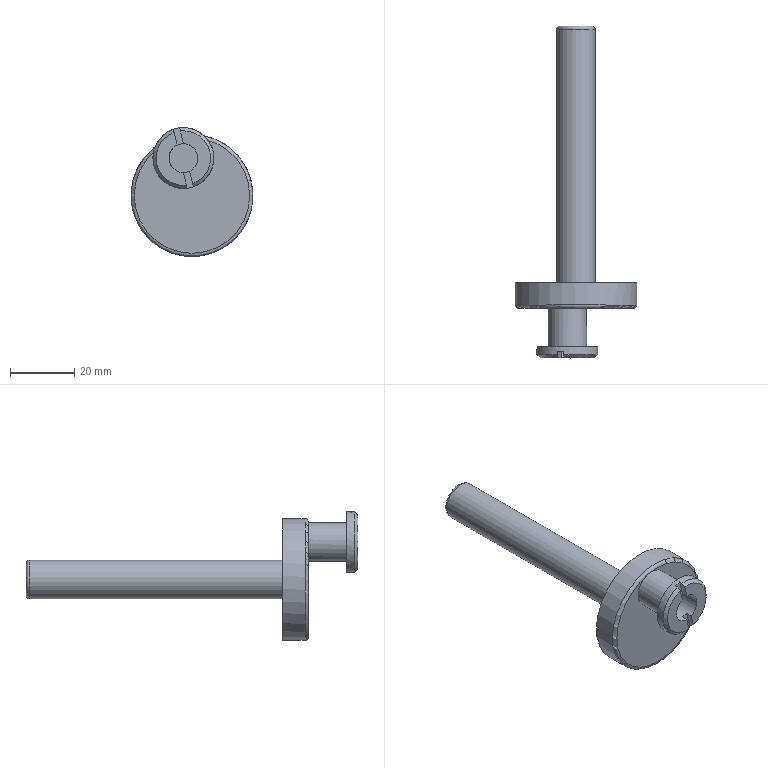Component | NX | CRANKSHAFT | 1 solid | 22 faces | volume 19607 mm3 | plane 13 | cylinder 5 | cone 2 | torus 2 | commonest cylinder face diameters 12 x2 19 x1 38 x1 9 x1